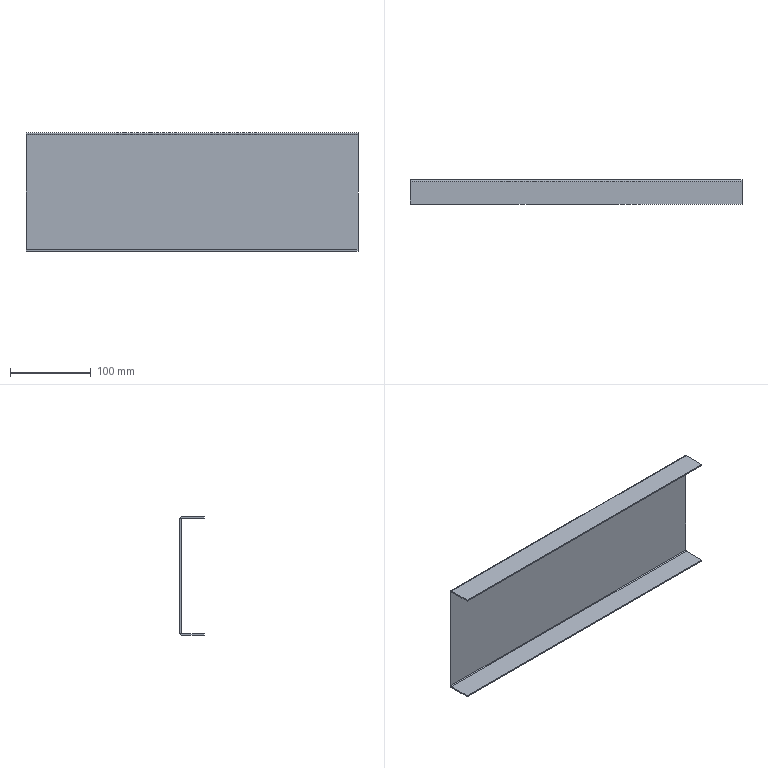Component | SolidWorks | HeatingBoxCover.1-1 | 1 solid | 22 faces | box 410 x 30 x 146 mm | volume 123921 mm3 | plane 18 | cylinder 4 | commonest cylinder face diameters 5 x2 2 x2
STEP:
#1=CARTESIAN_POINT('',(5.,5.315,-2.672));
#2=VERTEX_POINT('',#1);
#3=CARTESIAN_POINT('',(5.,5.256,-2.672));
#4=VERTEX_POINT('',#3);
#5=CARTESIAN_POINT('',(5.,5.315,-2.672));
#6=DIRECTION('',(-0.,-1.,0.));
#7=VECTOR('',#6,39.37);
#8=LINE('',#5,#7);
#9=EDGE_CURVE('',#2,#4,#8,.T.);
#10=ORIENTED_EDGE('',*,*,#9,.F.);
#11=CARTESIAN_POINT('',(5.,5.217,-2.771));
#12=VERTEX_POINT('',#11);
#13=CARTESIAN_POINT('',(5.,5.217,-2.672));
#14=DIRECTION('',(1.,-0.,0.));
#15=DIRECTION('',(0.,0.,1.));
#16=AXIS2_PLACEMENT_3D('',#13,#14,#15);
#17=CIRCLE('',#16,0.09843);
#18=EDGE_CURVE('',#12,#2,#17,.T.);
#19=ORIENTED_EDGE('',*,*,#18,.F.);
#20=CARTESIAN_POINT('',(5.,5.217,-2.712));
#21=VERTEX_POINT('',#20);
#22=CARTESIAN_POINT('',(5.,5.217,-2.712));
#23=DIRECTION('',(0.,0.,-1.));
#24=VECTOR('',#23,39.37);
#25=LINE('',#22,#24);
#26=EDGE_CURVE('',#21,#12,#25,.T.);
#27=ORIENTED_EDGE('',*,*,#26,.F.);
#28=CARTESIAN_POINT('',(5.,5.217,-2.672));
#29=DIRECTION('',(1.,-0.,0.));
#30=DIRECTION('',(0.,0.,1.));
#31=AXIS2_PLACEMENT_3D('',#28,#29,#30);
#32=CIRCLE('',#31,0.03937);
#33=EDGE_CURVE('',#21,#4,#32,.T.);
#34=ORIENTED_EDGE('',*,*,#33,.T.);
#35=EDGE_LOOP('',(#10,#19,#27,#34));
#36=FACE_OUTER_BOUND('',#35,.T.);
#37=CARTESIAN_POINT('',(5.,5.315,-2.672));
#38=DIRECTION('',(-1.,0.,-0.));
#39=DIRECTION('',(-0.,0.,1.));
#40=AXIS2_PLACEMENT_3D('',#37,#38,#39);
#41=PLANE('',#40);
#42=ADVANCED_FACE('',(#36),#41,.T.);
#43=CARTESIAN_POINT('',(5.,5.315,2.879));
#44=VERTEX_POINT('',#43);
#45=CARTESIAN_POINT('',(5.,5.315,2.977));
#46=DIRECTION('',(-0.,0.,1.));
#47=VECTOR('',#46,39.37);
#48=LINE('',#45,#47);
#49=EDGE_CURVE('',#2,#44,#48,.T.);
#50=ORIENTED_EDGE('',*,*,#49,.F.);
#51=ORIENTED_EDGE('',*,*,#9,.T.);
#52=CARTESIAN_POINT('',(5.,5.256,2.879));
#53=VERTEX_POINT('',#52);
#54=CARTESIAN_POINT('',(5.,5.256,2.977));
#55=DIRECTION('',(-0.,0.,1.));
#56=VECTOR('',#55,39.37);
#57=LINE('',#54,#56);
#58=EDGE_CURVE('',#4,#53,#57,.T.);
#59=ORIENTED_EDGE('',*,*,#58,.T.);
#60=CARTESIAN_POINT('',(5.,5.256,2.879));
#61=DIRECTION('',(0.,1.,-0.));
#62=VECTOR('',#61,39.37);
#63=LINE('',#60,#62);
#64=EDGE_CURVE('',#53,#44,#63,.T.);
#65=ORIENTED_EDGE('',*,*,#64,.T.);
#66=EDGE_LOOP('',(#50,#51,#59,#65));
#67=FACE_OUTER_BOUND('',#66,.T.);
#68=CARTESIAN_POINT('',(5.,5.217,-2.712));
#69=DIRECTION('',(-1.,0.,-0.));
#70=DIRECTION('',(-0.,0.,1.));
#71=AXIS2_PLACEMENT_3D('',#68,#69,#70);
#72=PLANE('',#71);
#73=ADVANCED_FACE('',(#67),#72,.T.);
#74=CARTESIAN_POINT('',(21.142,5.217,-2.771));
#75=VERTEX_POINT('',#74);
#76=CARTESIAN_POINT('',(21.142,5.217,-2.712));
#77=VERTEX_POINT('',#76);
#78=CARTESIAN_POINT('',(21.142,5.217,-2.771));
#79=DIRECTION('',(-0.,-0.,1.));
#80=VECTOR('',#79,39.37);
#81=LINE('',#78,#80);
#82=EDGE_CURVE('',#75,#77,#81,.T.);
#83=ORIENTED_EDGE('',*,*,#82,.F.);
#84=CARTESIAN_POINT('',(21.142,5.315,-2.672));
#85=VERTEX_POINT('',#84);
#86=CARTESIAN_POINT('',(21.142,5.217,-2.672));
#87=DIRECTION('',(1.,-0.,0.));
#88=DIRECTION('',(0.,0.,1.));
#89=AXIS2_PLACEMENT_3D('',#86,#87,#88);
#90=CIRCLE('',#89,0.09843);
#91=EDGE_CURVE('',#75,#85,#90,.T.);
#92=ORIENTED_EDGE('',*,*,#91,.T.);
#93=CARTESIAN_POINT('',(21.142,5.256,-2.672));
#94=VERTEX_POINT('',#93);
#95=CARTESIAN_POINT('',(21.142,5.256,-2.672));
#96=DIRECTION('',(0.,1.,-0.));
#97=VECTOR('',#96,39.37);
#98=LINE('',#95,#97);
#99=EDGE_CURVE('',#94,#85,#98,.T.);
#100=ORIENTED_EDGE('',*,*,#99,.F.);
#101=CARTESIAN_POINT('',(21.142,5.217,-2.672));
#102=DIRECTION('',(1.,-0.,0.));
#103=DIRECTION('',(0.,0.,1.));
#104=AXIS2_PLACEMENT_3D('',#101,#102,#103);
#105=CIRCLE('',#104,0.03937);
#106=EDGE_CURVE('',#77,#94,#105,.T.);
#107=ORIENTED_EDGE('',*,*,#106,.F.);
#108=EDGE_LOOP('',(#83,#92,#100,#107));
#109=FACE_OUTER_BOUND('',#108,.T.);
#110=CARTESIAN_POINT('',(21.142,5.217,-2.771));
#111=DIRECTION('',(1.,-0.,0.));
#112=DIRECTION('',(0.,-0.,-1.));
#113=AXIS2_PLACEMENT_3D('',#110,#111,#112);
#114=PLANE('',#113);
#115=ADVANCED_FACE('',(#109),#114,.T.);
#116=CARTESIAN_POINT('',(21.142,4.134,-2.771));
#117=VERTEX_POINT('',#116);
#118=CARTESIAN_POINT('',(21.142,5.315,-2.771));
#119=DIRECTION('',(0.,1.,-0.));
#120=VECTOR('',#119,39.37);
#121=LINE('',#118,#120);
#122=EDGE_CURVE('',#117,#75,#121,.T.);
#123=ORIENTED_EDGE('',*,*,#122,.T.);
#124=ORIENTED_EDGE('',*,*,#82,.T.);
#125=CARTESIAN_POINT('',(21.142,4.134,-2.712));
#126=VERTEX_POINT('',#125);
#127=CARTESIAN_POINT('',(21.142,5.315,-2.712));
#128=DIRECTION('',(0.,1.,-0.));
#129=VECTOR('',#128,39.37);
#130=LINE('',#127,#129);
#131=EDGE_CURVE('',#126,#77,#130,.T.);
#132=ORIENTED_EDGE('',*,*,#131,.F.);
#133=CARTESIAN_POINT('',(21.142,4.134,-2.712));
#134=DIRECTION('',(0.,-0.,-1.));
#135=VECTOR('',#134,39.37);
#136=LINE('',#133,#135);
#137=EDGE_CURVE('',#126,#117,#136,.T.);
#138=ORIENTED_EDGE('',*,*,#137,.T.);
#139=EDGE_LOOP('',(#123,#124,#132,#138));
#140=FACE_OUTER_BOUND('',#139,.T.);
#141=CARTESIAN_POINT('',(21.142,5.256,-2.672));
#142=DIRECTION('',(1.,-0.,0.));
#143=DIRECTION('',(0.,-0.,-1.));
#144=AXIS2_PLACEMENT_3D('',#141,#142,#143);
#145=PLANE('',#144);
#146=ADVANCED_FACE('',(#140),#145,.T.);
#147=CARTESIAN_POINT('',(5.,5.217,2.977));
#148=VERTEX_POINT('',#147);
#149=CARTESIAN_POINT('',(5.,5.217,2.918));
#150=VERTEX_POINT('',#149);
#151=CARTESIAN_POINT('',(5.,5.217,2.977));
#152=DIRECTION('',(0.,-0.,-1.));
#153=VECTOR('',#152,39.37);
#154=LINE('',#151,#153);
#155=EDGE_CURVE('',#148,#150,#154,.T.);
#156=ORIENTED_EDGE('',*,*,#155,.F.);
#157=CARTESIAN_POINT('',(5.,5.217,2.879));
#158=DIRECTION('',(1.,-0.,0.));
#159=DIRECTION('',(0.,0.,1.));
#160=AXIS2_PLACEMENT_3D('',#157,#158,#159);
#161=CIRCLE('',#160,0.09843);
#162=EDGE_CURVE('',#44,#148,#161,.T.);
#163=ORIENTED_EDGE('',*,*,#162,.F.);
#164=ORIENTED_EDGE('',*,*,#64,.F.);
#165=CARTESIAN_POINT('',(5.,5.217,2.879));
#166=DIRECTION('',(1.,-0.,0.));
#167=DIRECTION('',(0.,0.,1.));
#168=AXIS2_PLACEMENT_3D('',#165,#166,#167);
#169=CIRCLE('',#168,0.03937);
#170=EDGE_CURVE('',#53,#150,#169,.T.);
#171=ORIENTED_EDGE('',*,*,#170,.T.);
#172=EDGE_LOOP('',(#156,#163,#164,#171));
#173=FACE_OUTER_BOUND('',#172,.T.);
#174=CARTESIAN_POINT('',(5.,5.217,2.977));
#175=DIRECTION('',(-1.,0.,-0.));
#176=DIRECTION('',(-0.,0.,1.));
#177=AXIS2_PLACEMENT_3D('',#174,#175,#176);
#178=PLANE('',#177);
#179=ADVANCED_FACE('',(#173),#178,.T.);
#180=CARTESIAN_POINT('',(5.,4.134,2.977));
#181=VERTEX_POINT('',#180);
#182=CARTESIAN_POINT('',(5.,5.315,2.977));
#183=DIRECTION('',(-0.,-1.,0.));
#184=VECTOR('',#183,39.37);
#185=LINE('',#182,#184);
#186=EDGE_CURVE('',#148,#181,#185,.T.);
#187=ORIENTED_EDGE('',*,*,#186,.F.);
#188=ORIENTED_EDGE('',*,*,#155,.T.);
#189=CARTESIAN_POINT('',(5.,4.134,2.918));
#190=VERTEX_POINT('',#189);
#191=CARTESIAN_POINT('',(5.,5.315,2.918));
#192=DIRECTION('',(-0.,-1.,0.));
#193=VECTOR('',#192,39.37);
#194=LINE('',#191,#193);
#195=EDGE_CURVE('',#150,#190,#194,.T.);
#196=ORIENTED_EDGE('',*,*,#195,.T.);
#197=CARTESIAN_POINT('',(5.,4.134,2.977));
#198=DIRECTION('',(0.,-0.,-1.));
#199=VECTOR('',#198,39.37);
#200=LINE('',#197,#199);
#201=EDGE_CURVE('',#181,#190,#200,.T.);
#202=ORIENTED_EDGE('',*,*,#201,.F.);
#203=EDGE_LOOP('',(#187,#188,#196,#202));
#204=FACE_OUTER_BOUND('',#203,.T.);
#205=CARTESIAN_POINT('',(5.,5.256,2.879));
#206=DIRECTION('',(-1.,0.,-0.));
#207=DIRECTION('',(-0.,0.,1.));
#208=AXIS2_PLACEMENT_3D('',#205,#206,#207);
#209=PLANE('',#208);
#210=ADVANCED_FACE('',(#204),#209,.T.);
#211=CARTESIAN_POINT('',(21.142,5.315,2.879));
#212=VERTEX_POINT('',#211);
#213=CARTESIAN_POINT('',(21.142,5.256,2.879));
#214=VERTEX_POINT('',#213);
#215=CARTESIAN_POINT('',(21.142,5.315,2.879));
#216=DIRECTION('',(-0.,-1.,0.));
#217=VECTOR('',#216,39.37);
#218=LINE('',#215,#217);
#219=EDGE_CURVE('',#212,#214,#218,.T.);
#220=ORIENTED_EDGE('',*,*,#219,.F.);
#221=CARTESIAN_POINT('',(21.142,5.217,2.977));
#222=VERTEX_POINT('',#221);
#223=CARTESIAN_POINT('',(21.142,5.217,2.879));
#224=DIRECTION('',(1.,-0.,0.));
#225=DIRECTION('',(0.,0.,1.));
#226=AXIS2_PLACEMENT_3D('',#223,#224,#225);
#227=CIRCLE('',#226,0.09843);
#228=EDGE_CURVE('',#212,#222,#227,.T.);
#229=ORIENTED_EDGE('',*,*,#228,.T.);
#230=CARTESIAN_POINT('',(21.142,5.217,2.918));
#231=VERTEX_POINT('',#230);
#232=CARTESIAN_POINT('',(21.142,5.217,2.918));
#233=DIRECTION('',(-0.,0.,1.));
#234=VECTOR('',#233,39.37);
#235=LINE('',#232,#234);
#236=EDGE_CURVE('',#231,#222,#235,.T.);
#237=ORIENTED_EDGE('',*,*,#236,.F.);
#238=CARTESIAN_POINT('',(21.142,5.217,2.879));
#239=DIRECTION('',(1.,-0.,0.));
#240=DIRECTION('',(0.,0.,1.));
#241=AXIS2_PLACEMENT_3D('',#238,#239,#240);
#242=CIRCLE('',#241,0.03937);
#243=EDGE_CURVE('',#214,#231,#242,.T.);
#244=ORIENTED_EDGE('',*,*,#243,.F.);
#245=EDGE_LOOP('',(#220,#229,#237,#244));
#246=FACE_OUTER_BOUND('',#245,.T.);
#247=CARTESIAN_POINT('',(21.142,5.315,2.879));
#248=DIRECTION('',(1.,-0.,0.));
#249=DIRECTION('',(0.,-0.,-1.));
#250=AXIS2_PLACEMENT_3D('',#247,#248,#249);
#251=PLANE('',#250);
#252=ADVANCED_FACE('',(#246),#251,.T.);
#253=CARTESIAN_POINT('',(21.142,5.315,2.977));
#254=DIRECTION('',(-0.,0.,1.));
#255=VECTOR('',#254,39.37);
#256=LINE('',#253,#255);
#257=EDGE_CURVE('',#85,#212,#256,.T.);
#258=ORIENTED_EDGE('',*,*,#257,.T.);
#259=ORIENTED_EDGE('',*,*,#219,.T.);
#260=CARTESIAN_POINT('',(21.142,5.256,2.977));
#261=DIRECTION('',(-0.,0.,1.));
#262=VECTOR('',#261,39.37);
#263=LINE('',#260,#262);
#264=EDGE_CURVE('',#94,#214,#263,.T.);
#265=ORIENTED_EDGE('',*,*,#264,.F.);
#266=ORIENTED_EDGE('',*,*,#99,.T.);
#267=EDGE_LOOP('',(#258,#259,#265,#266));
#268=FACE_OUTER_BOUND('',#267,.T.);
#269=CARTESIAN_POINT('',(21.142,5.217,2.918));
#270=DIRECTION('',(1.,-0.,0.));
#271=DIRECTION('',(0.,-0.,-1.));
#272=AXIS2_PLACEMENT_3D('',#269,#270,#271);
#273=PLANE('',#272);
#274=ADVANCED_FACE('',(#268),#273,.T.);
#275=CARTESIAN_POINT('',(21.142,4.134,2.918));
#276=VERTEX_POINT('',#275);
#277=CARTESIAN_POINT('',(21.142,5.315,2.918));
#278=DIRECTION('',(-0.,-1.,0.));
#279=VECTOR('',#278,39.37);
#280=LINE('',#277,#279);
#281=EDGE_CURVE('',#231,#276,#280,.T.);
#282=ORIENTED_EDGE('',*,*,#281,.T.);
#283=CARTESIAN_POINT('',(5.,4.134,2.918));
#284=DIRECTION('',(1.,-0.,0.));
#285=VECTOR('',#284,39.37);
#286=LINE('',#283,#285);
#287=EDGE_CURVE('',#190,#276,#286,.T.);
#288=ORIENTED_EDGE('',*,*,#287,.F.);
#289=ORIENTED_EDGE('',*,*,#195,.F.);
#290=CARTESIAN_POINT('',(5.,5.217,2.918));
#291=DIRECTION('',(1.,-0.,0.));
#292=VECTOR('',#291,39.37);
#293=LINE('',#290,#292);
#294=EDGE_CURVE('',#150,#231,#293,.T.);
#295=ORIENTED_EDGE('',*,*,#294,.T.);
#296=EDGE_LOOP('',(#282,#288,#289,#295));
#297=FACE_OUTER_BOUND('',#296,.T.);
#298=CARTESIAN_POINT('',(5.,5.315,2.918));
#299=DIRECTION('',(-0.,0.,1.));
#300=DIRECTION('',(1.,-0.,0.));
#301=AXIS2_PLACEMENT_3D('',#298,#299,#300);
#302=PLANE('',#301);
#303=ADVANCED_FACE('',(#297),#302,.F.);
#304=CARTESIAN_POINT('',(21.142,4.134,2.977));
#305=VERTEX_POINT('',#304);
#306=CARTESIAN_POINT('',(21.142,4.134,2.977));
#307=DIRECTION('',(0.,-0.,-1.));
#308=VECTOR('',#307,39.37);
#309=LINE('',#306,#308);
#310=EDGE_CURVE('',#305,#276,#309,.T.);
#311=ORIENTED_EDGE('',*,*,#310,.F.);
#312=CARTESIAN_POINT('',(5.,4.134,2.977));
#313=DIRECTION('',(1.,-0.,0.));
#314=VECTOR('',#313,39.37);
#315=LINE('',#312,#314);
#316=EDGE_CURVE('',#181,#305,#315,.T.);
#317=ORIENTED_EDGE('',*,*,#316,.F.);
#318=ORIENTED_EDGE('',*,*,#201,.T.);
#319=ORIENTED_EDGE('',*,*,#287,.T.);
#320=EDGE_LOOP('',(#311,#317,#318,#319));
#321=FACE_OUTER_BOUND('',#320,.T.);
#322=CARTESIAN_POINT('',(5.,4.134,2.977));
#323=DIRECTION('',(-0.,-1.,0.));
#324=DIRECTION('',(1.,-0.,0.));
#325=AXIS2_PLACEMENT_3D('',#322,#323,#324);
#326=PLANE('',#325);
#327=ADVANCED_FACE('',(#321),#326,.T.);
#328=CARTESIAN_POINT('',(21.142,5.315,2.977));
#329=DIRECTION('',(-0.,-1.,0.));
#330=VECTOR('',#329,39.37);
#331=LINE('',#328,#330);
#332=EDGE_CURVE('',#222,#305,#331,.T.);
#333=ORIENTED_EDGE('',*,*,#332,.F.);
#334=CARTESIAN_POINT('',(5.,5.217,2.977));
#335=DIRECTION('',(1.,-0.,0.));
#336=VECTOR('',#335,39.37);
#337=LINE('',#334,#336);
#338=EDGE_CURVE('',#148,#222,#337,.T.);
#339=ORIENTED_EDGE('',*,*,#338,.F.);
#340=ORIENTED_EDGE('',*,*,#186,.T.);
#341=ORIENTED_EDGE('',*,*,#316,.T.);
#342=EDGE_LOOP('',(#333,#339,#340,#341));
#343=FACE_OUTER_BOUND('',#342,.T.);
#344=CARTESIAN_POINT('',(5.,5.315,2.977));
#345=DIRECTION('',(-0.,0.,1.));
#346=DIRECTION('',(1.,-0.,0.));
#347=AXIS2_PLACEMENT_3D('',#344,#345,#346);
#348=PLANE('',#347);
#349=ADVANCED_FACE('',(#343),#348,.T.);
#350=ORIENTED_EDGE('',*,*,#228,.F.);
#351=CARTESIAN_POINT('',(5.,5.315,2.879));
#352=DIRECTION('',(1.,-0.,0.));
#353=VECTOR('',#352,39.37);
#354=LINE('',#351,#353);
#355=EDGE_CURVE('',#44,#212,#354,.T.);
#356=ORIENTED_EDGE('',*,*,#355,.F.);
#357=ORIENTED_EDGE('',*,*,#162,.T.);
#358=ORIENTED_EDGE('',*,*,#338,.T.);
#359=EDGE_LOOP('',(#350,#356,#357,#358));
#360=FACE_OUTER_BOUND('',#359,.T.);
#361=CARTESIAN_POINT('',(5.,5.217,2.879));
#362=DIRECTION('',(1.,-0.,0.));
#363=DIRECTION('',(0.,0.,-1.));
#364=AXIS2_PLACEMENT_3D('',#361,#362,#363);
#365=CYLINDRICAL_SURFACE('',#364,0.09843);
#366=ADVANCED_FACE('',(#360),#365,.T.);
#367=ORIENTED_EDGE('',*,*,#257,.F.);
#368=CARTESIAN_POINT('',(5.,5.315,-2.672));
#369=DIRECTION('',(1.,-0.,0.));
#370=VECTOR('',#369,39.37);
#371=LINE('',#368,#370);
#372=EDGE_CURVE('',#2,#85,#371,.T.);
#373=ORIENTED_EDGE('',*,*,#372,.F.);
#374=ORIENTED_EDGE('',*,*,#49,.T.);
#375=ORIENTED_EDGE('',*,*,#355,.T.);
#376=EDGE_LOOP('',(#367,#373,#374,#375));
#377=FACE_OUTER_BOUND('',#376,.T.);
#378=CARTESIAN_POINT('',(5.,5.315,2.977));
#379=DIRECTION('',(0.,1.,-0.));
#380=DIRECTION('',(0.,-0.,-1.));
#381=AXIS2_PLACEMENT_3D('',#378,#379,#380);
#382=PLANE('',#381);
#383=ADVANCED_FACE('',(#377),#382,.T.);
#384=ORIENTED_EDGE('',*,*,#91,.F.);
#385=CARTESIAN_POINT('',(5.,5.217,-2.771));
#386=DIRECTION('',(1.,-0.,0.));
#387=VECTOR('',#386,39.37);
#388=LINE('',#385,#387);
#389=EDGE_CURVE('',#12,#75,#388,.T.);
#390=ORIENTED_EDGE('',*,*,#389,.F.);
#391=ORIENTED_EDGE('',*,*,#18,.T.);
#392=ORIENTED_EDGE('',*,*,#372,.T.);
#393=EDGE_LOOP('',(#384,#390,#391,#392));
#394=FACE_OUTER_BOUND('',#393,.T.);
#395=CARTESIAN_POINT('',(5.,5.217,-2.672));
#396=DIRECTION('',(1.,-0.,0.));
#397=DIRECTION('',(0.,0.,-1.));
#398=AXIS2_PLACEMENT_3D('',#395,#396,#397);
#399=CYLINDRICAL_SURFACE('',#398,0.09843);
#400=ADVANCED_FACE('',(#394),#399,.T.);
#401=ORIENTED_EDGE('',*,*,#122,.F.);
#402=CARTESIAN_POINT('',(5.,4.134,-2.771));
#403=VERTEX_POINT('',#402);
#404=CARTESIAN_POINT('',(5.,4.134,-2.771));
#405=DIRECTION('',(1.,-0.,0.));
#406=VECTOR('',#405,39.37);
#407=LINE('',#404,#406);
#408=EDGE_CURVE('',#403,#117,#407,.T.);
#409=ORIENTED_EDGE('',*,*,#408,.F.);
#410=CARTESIAN_POINT('',(5.,5.315,-2.771));
#411=DIRECTION('',(0.,1.,-0.));
#412=VECTOR('',#411,39.37);
#413=LINE('',#410,#412);
#414=EDGE_CURVE('',#403,#12,#413,.T.);
#415=ORIENTED_EDGE('',*,*,#414,.T.);
#416=ORIENTED_EDGE('',*,*,#389,.T.);
#417=EDGE_LOOP('',(#401,#409,#415,#416));
#418=FACE_OUTER_BOUND('',#417,.T.);
#419=CARTESIAN_POINT('',(5.,5.315,-2.771));
#420=DIRECTION('',(0.,-0.,-1.));
#421=DIRECTION('',(-1.,0.,-0.));
#422=AXIS2_PLACEMENT_3D('',#419,#420,#421);
#423=PLANE('',#422);
#424=ADVANCED_FACE('',(#418),#423,.T.);
#425=ORIENTED_EDGE('',*,*,#137,.F.);
#426=CARTESIAN_POINT('',(5.,4.134,-2.712));
#427=VERTEX_POINT('',#426);
#428=CARTESIAN_POINT('',(5.,4.134,-2.712));
#429=DIRECTION('',(1.,-0.,0.));
#430=VECTOR('',#429,39.37);
#431=LINE('',#428,#430);
#432=EDGE_CURVE('',#427,#126,#431,.T.);
#433=ORIENTED_EDGE('',*,*,#432,.F.);
#434=CARTESIAN_POINT('',(5.,4.134,-2.712));
#435=DIRECTION('',(0.,-0.,-1.));
#436=VECTOR('',#435,39.37);
#437=LINE('',#434,#436);
#438=EDGE_CURVE('',#427,#403,#437,.T.);
#439=ORIENTED_EDGE('',*,*,#438,.T.);
#440=ORIENTED_EDGE('',*,*,#408,.T.);
#441=EDGE_LOOP('',(#425,#433,#439,#440));
#442=FACE_OUTER_BOUND('',#441,.T.);
#443=CARTESIAN_POINT('',(5.,4.134,-2.712));
#444=DIRECTION('',(-0.,-1.,0.));
#445=DIRECTION('',(1.,-0.,0.));
#446=AXIS2_PLACEMENT_3D('',#443,#444,#445);
#447=PLANE('',#446);
#448=ADVANCED_FACE('',(#442),#447,.T.);
#449=ORIENTED_EDGE('',*,*,#131,.T.);
#450=CARTESIAN_POINT('',(5.,5.217,-2.712));
#451=DIRECTION('',(1.,-0.,0.));
#452=VECTOR('',#451,39.37);
#453=LINE('',#450,#452);
#454=EDGE_CURVE('',#21,#77,#453,.T.);
#455=ORIENTED_EDGE('',*,*,#454,.F.);
#456=CARTESIAN_POINT('',(5.,5.315,-2.712));
#457=DIRECTION('',(0.,1.,-0.));
#458=VECTOR('',#457,39.37);
#459=LINE('',#456,#458);
#460=EDGE_CURVE('',#427,#21,#459,.T.);
#461=ORIENTED_EDGE('',*,*,#460,.F.);
#462=ORIENTED_EDGE('',*,*,#432,.T.);
#463=EDGE_LOOP('',(#449,#455,#461,#462));
#464=FACE_OUTER_BOUND('',#463,.T.);
#465=CARTESIAN_POINT('',(5.,5.315,-2.712));
#466=DIRECTION('',(0.,-0.,-1.));
#467=DIRECTION('',(-1.,0.,-0.));
#468=AXIS2_PLACEMENT_3D('',#465,#466,#467);
#469=PLANE('',#468);
#470=ADVANCED_FACE('',(#464),#469,.F.);
#471=ORIENTED_EDGE('',*,*,#106,.T.);
#472=CARTESIAN_POINT('',(5.,5.256,-2.672));
#473=DIRECTION('',(1.,-0.,0.));
#474=VECTOR('',#473,39.37);
#475=LINE('',#472,#474);
#476=EDGE_CURVE('',#4,#94,#475,.T.);
#477=ORIENTED_EDGE('',*,*,#476,.F.);
#478=ORIENTED_EDGE('',*,*,#33,.F.);
#479=ORIENTED_EDGE('',*,*,#454,.T.);
#480=EDGE_LOOP('',(#471,#477,#478,#479));
#481=FACE_OUTER_BOUND('',#480,.T.);
#482=CARTESIAN_POINT('',(5.,5.217,-2.672));
#483=DIRECTION('',(1.,-0.,0.));
#484=DIRECTION('',(0.,0.,-1.));
#485=AXIS2_PLACEMENT_3D('',#482,#483,#484);
#486=CYLINDRICAL_SURFACE('',#485,0.03937);
#487=ADVANCED_FACE('',(#481),#486,.F.);
#488=ORIENTED_EDGE('',*,*,#264,.T.);
#489=CARTESIAN_POINT('',(5.,5.256,2.879));
#490=DIRECTION('',(1.,-0.,0.));
#491=VECTOR('',#490,39.37);
#492=LINE('',#489,#491);
#493=EDGE_CURVE('',#53,#214,#492,.T.);
#494=ORIENTED_EDGE('',*,*,#493,.F.);
#495=ORIENTED_EDGE('',*,*,#58,.F.);
#496=ORIENTED_EDGE('',*,*,#476,.T.);
#497=EDGE_LOOP('',(#488,#494,#495,#496));
#498=FACE_OUTER_BOUND('',#497,.T.);
#499=CARTESIAN_POINT('',(5.,5.256,2.977));
#500=DIRECTION('',(0.,1.,-0.));
#501=DIRECTION('',(0.,-0.,-1.));
#502=AXIS2_PLACEMENT_3D('',#499,#500,#501);
#503=PLANE('',#502);
#504=ADVANCED_FACE('',(#498),#503,.F.);
#505=ORIENTED_EDGE('',*,*,#243,.T.);
#506=ORIENTED_EDGE('',*,*,#294,.F.);
#507=ORIENTED_EDGE('',*,*,#170,.F.);
#508=ORIENTED_EDGE('',*,*,#493,.T.);
#509=EDGE_LOOP('',(#505,#506,#507,#508));
#510=FACE_OUTER_BOUND('',#509,.T.);
#511=CARTESIAN_POINT('',(5.,5.217,2.879));
#512=DIRECTION('',(1.,-0.,0.));
#513=DIRECTION('',(0.,0.,-1.));
#514=AXIS2_PLACEMENT_3D('',#511,#512,#513);
#515=CYLINDRICAL_SURFACE('',#514,0.03937);
#516=ADVANCED_FACE('',(#510),#515,.F.);
#517=ORIENTED_EDGE('',*,*,#460,.T.);
#518=ORIENTED_EDGE('',*,*,#26,.T.);
#519=ORIENTED_EDGE('',*,*,#414,.F.);
#520=ORIENTED_EDGE('',*,*,#438,.F.);
#521=EDGE_LOOP('',(#517,#518,#519,#520));
#522=FACE_OUTER_BOUND('',#521,.T.);
#523=CARTESIAN_POINT('',(5.,5.217,2.879));
#524=DIRECTION('',(-1.,0.,-0.));
#525=DIRECTION('',(-0.,0.,1.));
#526=AXIS2_PLACEMENT_3D('',#523,#524,#525);
#527=PLANE('',#526);
#528=ADVANCED_FACE('',(#522),#527,.T.);
#529=ORIENTED_EDGE('',*,*,#281,.F.);
#530=ORIENTED_EDGE('',*,*,#236,.T.);
#531=ORIENTED_EDGE('',*,*,#332,.T.);
#532=ORIENTED_EDGE('',*,*,#310,.T.);
#533=EDGE_LOOP('',(#529,#530,#531,#532));
#534=FACE_OUTER_BOUND('',#533,.T.);
#535=CARTESIAN_POINT('',(21.142,5.217,2.879));
#536=DIRECTION('',(-1.,0.,-0.));
#537=DIRECTION('',(-0.,0.,1.));
#538=AXIS2_PLACEMENT_3D('',#535,#536,#537);
#539=PLANE('',#538);
#540=ADVANCED_FACE('',(#534),#539,.F.);
#541=CLOSED_SHELL('',(#42,#73,#115,#146,#179,#210,#252,#274,#303,#327,#349,#366,#383,#400,#424,#448,#470,#487,#504,#516,#528,#540));
#542=MANIFOLD_SOLID_BREP('',#541);
#543=CARTESIAN_POINT('',(0.,0.,0.));
#544=DIRECTION('',(0.,0.,1.));
#545=DIRECTION('',(1.,0.,0.));
#546=AXIS2_PLACEMENT_3D('',#543,#544,#545);
#547=(LENGTH_UNIT()NAMED_UNIT(*)SI_UNIT($,.METRE.));
#548=LENGTH_MEASURE_WITH_UNIT(LENGTH_MEASURE(0.0254),#547);
#549=DIMENSIONAL_EXPONENTS(1.,0.,0.,0.,0.,0.,0.);
#550=(CONVERSION_BASED_UNIT('',#548)LENGTH_UNIT()NAMED_UNIT(#549));
#551=UNCERTAINTY_MEASURE_WITH_UNIT(LENGTH_MEASURE(0.00001),#550,'','');
#552=(NAMED_UNIT(*)PLANE_ANGLE_UNIT()SI_UNIT($,.RADIAN.));
#553=(NAMED_UNIT(*)SI_UNIT($,.STERADIAN.)SOLID_ANGLE_UNIT());
#554=(GEOMETRIC_REPRESENTATION_CONTEXT(3)GLOBAL_UNCERTAINTY_ASSIGNED_CONTEXT((#551))GLOBAL_UNIT_ASSIGNED_CONTEXT((#550,#552,#553))REPRESENTATION_CONTEXT('',''));
#555=ADVANCED_BREP_SHAPE_REPRESENTATION('',(#542,#546),#554);
#556=COLOUR_RGB('',0.7922,0.8196,0.9333);
#557=FILL_AREA_STYLE_COLOUR('',#556);
#558=FILL_AREA_STYLE('',(#557));
#559=SURFACE_STYLE_FILL_AREA(#558);
#560=SURFACE_SIDE_STYLE('',(#559));
#561=SURFACE_STYLE_USAGE(.BOTH.,#560);
#562=PRESENTATION_STYLE_ASSIGNMENT((#561));
#563=STYLED_ITEM('',(#562),#542);
#564=PRESENTATION_LAYER_ASSIGNMENT('','',(#563));
#565=(LENGTH_UNIT()NAMED_UNIT(*)SI_UNIT($,.METRE.));
#566=LENGTH_MEASURE_WITH_UNIT(LENGTH_MEASURE(0.0254),#565);
#567=DIMENSIONAL_EXPONENTS(1.,0.,0.,0.,0.,0.,0.);
#568=(CONVERSION_BASED_UNIT('',#566)LENGTH_UNIT()NAMED_UNIT(#567));
#569=UNCERTAINTY_MEASURE_WITH_UNIT(LENGTH_MEASURE(0.00001),#568,'','');
#570=(NAMED_UNIT(*)PLANE_ANGLE_UNIT()SI_UNIT($,.RADIAN.));
#571=(NAMED_UNIT(*)SI_UNIT($,.STERADIAN.)SOLID_ANGLE_UNIT());
#572=(GEOMETRIC_REPRESENTATION_CONTEXT(3)GLOBAL_UNCERTAINTY_ASSIGNED_CONTEXT((#569))GLOBAL_UNIT_ASSIGNED_CONTEXT((#568,#570,#571))REPRESENTATION_CONTEXT('',''));
#573=MECHANICAL_DESIGN_GEOMETRIC_PRESENTATION_REPRESENTATION('',(#563),#572);